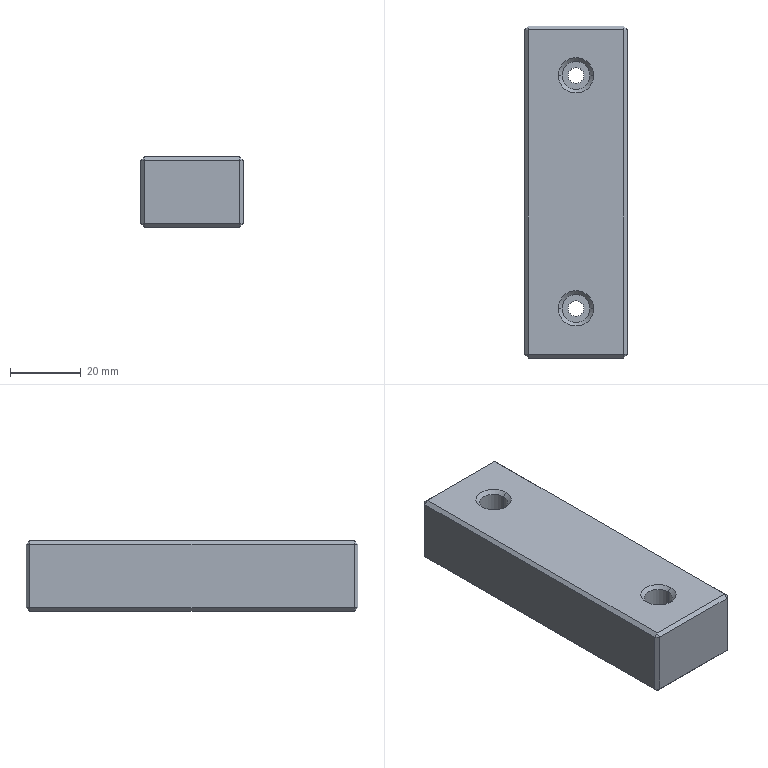Component | SolidWorks | CutterNylonPad-1 | 1 solid | 44 faces | box 29 x 94 x 20 mm | volume 52529 mm3 | plane 28 | cone 8 | cylinder 8 | commonest cylinder face diameters 8 x4 4.5 x4 | material 1060 Alloy
build123d program:
from build123d import *

# Parameters (mm, degrees)
SKETCH1_W                                          = 94
SKETCH1_H                                          = 20
BOSS_EXTRUDE1_DEPTH                                = 14.5
HOLE_SIZE_ACCORDING_TO_TYPE_OF_HEXAGON_D           = 4.5
HOLE_SIZE_ACCORDING_TO_TYPE_OF_HEXAGON_CBORE_D     = 8
HOLE_SIZE_ACCORDING_TO_TYPE_OF_HEXAGON_CBORE_DEPTH = 15
CHAMFER1_SIZE                                      = 1


with BuildPart() as part:
    # Sketch1 → Boss-Extrude1 (new, symmetric)
    with BuildSketch(Plane.XY):
        with Locations((0, -10)):
            Rectangle(SKETCH1_W, SKETCH1_H)
    extrude(amount=BOSS_EXTRUDE1_DEPTH, both=True)

    # Hole Size_ according to_Type of Hexagon (through all)
    with Locations(Plane(origin=(0, 0, 0), x_dir=(1, 0, 0), z_dir=(0, 1, 0))):
        with Locations((-33, 0), (33, 0)):
            CounterBoreHole(HOLE_SIZE_ACCORDING_TO_TYPE_OF_HEXAGON_D / 2, HOLE_SIZE_ACCORDING_TO_TYPE_OF_HEXAGON_CBORE_D / 2, HOLE_SIZE_ACCORDING_TO_TYPE_OF_HEXAGON_CBORE_DEPTH)

    # Chamfer1
    chamfer1_edges = [part.edges().sort_by_distance(p)[0] for p in [
        (47, -10, 14.5),
        (0, 0, 14.5),
        (29, 0, 0),
        (35.25, -20, 0),
        (-37, 0, 0),
        (-30.75, -20, 0),
        (-47, -10, 14.5),
        (0, 0, -14.5),
        (47, -10, -14.5),
        (0, -20, -14.5),
        (-47, -10, -14.5),
        (0, -20, 14.5),
        (-47, 0, 0),
        (47, 0, 0),
        (47, -20, 0),
        (-47, -20, 0),
    ]]
    chamfer(chamfer1_edges, length=CHAMFER1_SIZE)


solid = part.part

# Placed as in the assembly
solid = solid.moved(Location((-194.766, 347.264, -17), (90, -90, 0)))
STEP:
#1=COLOUR_RGB('',0.7922,0.8196,0.9333);
#2=FILL_AREA_STYLE_COLOUR('',#1);
#3=FILL_AREA_STYLE('',(#2));
#4=SURFACE_STYLE_FILL_AREA(#3);
#5=SURFACE_SIDE_STYLE('',(#4));
#6=SURFACE_STYLE_USAGE(.BOTH.,#5);
#7=PRESENTATION_STYLE_ASSIGNMENT((#6));
#8=CARTESIAN_POINT('',(-7.825,12.373,-0.7087));
#9=VERTEX_POINT('',#8);
#10=CARTESIAN_POINT('',(-7.51,12.373,-0.7087));
#11=VERTEX_POINT('',#10);
#12=CARTESIAN_POINT('',(-7.668,12.373,-0.7087));
#13=DIRECTION('',(-0.,-0.,1.));
#14=DIRECTION('',(-1.,0.,0.));
#15=AXIS2_PLACEMENT_3D('',#12,#13,#14);
#16=CIRCLE('',#15,0.1575);
#17=EDGE_CURVE('',#9,#11,#16,.T.);
#18=ORIENTED_EDGE('',*,*,#17,.F.);
#19=CARTESIAN_POINT('',(-7.865,12.373,-0.6693));
#20=VERTEX_POINT('',#19);
#21=CARTESIAN_POINT('',(-7.825,12.373,-0.7087));
#22=DIRECTION('',(-0.7071,0.,0.7071));
#23=VECTOR('',#22,39.37);
#24=LINE('',#21,#23);
#25=EDGE_CURVE('',#9,#20,#24,.T.);
#26=ORIENTED_EDGE('',*,*,#25,.T.);
#27=CARTESIAN_POINT('',(-7.471,12.373,-0.6693));
#28=VERTEX_POINT('',#27);
#29=CARTESIAN_POINT('',(-7.668,12.373,-0.6693));
#30=DIRECTION('',(0.,0.,-1.));
#31=DIRECTION('',(-1.,0.,0.));
#32=AXIS2_PLACEMENT_3D('',#29,#30,#31);
#33=CIRCLE('',#32,0.1969);
#34=EDGE_CURVE('',#28,#20,#33,.T.);
#35=ORIENTED_EDGE('',*,*,#34,.F.);
#36=CARTESIAN_POINT('',(-7.51,12.373,-0.7087));
#37=DIRECTION('',(0.7071,-0.,0.7071));
#38=VECTOR('',#37,39.37);
#39=LINE('',#36,#38);
#40=EDGE_CURVE('',#11,#28,#39,.T.);
#41=ORIENTED_EDGE('',*,*,#40,.F.);
#42=EDGE_LOOP('',(#18,#26,#35,#41));
#43=FACE_OUTER_BOUND('',#42,.T.);
#44=CARTESIAN_POINT('',(-7.668,12.373,-0.7087));
#45=DIRECTION('',(-0.,-0.,1.));
#46=DIRECTION('',(1.,0.,0.));
#47=AXIS2_PLACEMENT_3D('',#44,#45,#46);
#48=CONICAL_SURFACE('',#47,0.1575,0.7854);
#49=ADVANCED_FACE('',(#43),#48,.F.);
#50=CARTESIAN_POINT('',(-7.825,14.971,-0.7087));
#51=VERTEX_POINT('',#50);
#52=CARTESIAN_POINT('',(-7.51,14.971,-0.7087));
#53=VERTEX_POINT('',#52);
#54=CARTESIAN_POINT('',(-7.668,14.971,-0.7087));
#55=DIRECTION('',(-0.,-0.,1.));
#56=DIRECTION('',(-1.,0.,0.));
#57=AXIS2_PLACEMENT_3D('',#54,#55,#56);
#58=CIRCLE('',#57,0.1575);
#59=EDGE_CURVE('',#51,#53,#58,.T.);
#60=ORIENTED_EDGE('',*,*,#59,.F.);
#61=CARTESIAN_POINT('',(-7.865,14.971,-0.6693));
#62=VERTEX_POINT('',#61);
#63=CARTESIAN_POINT('',(-7.825,14.971,-0.7087));
#64=DIRECTION('',(-0.7071,0.,0.7071));
#65=VECTOR('',#64,39.37);
#66=LINE('',#63,#65);
#67=EDGE_CURVE('',#51,#62,#66,.T.);
#68=ORIENTED_EDGE('',*,*,#67,.T.);
#69=CARTESIAN_POINT('',(-7.471,14.971,-0.6693));
#70=VERTEX_POINT('',#69);
#71=CARTESIAN_POINT('',(-7.668,14.971,-0.6693));
#72=DIRECTION('',(0.,0.,-1.));
#73=DIRECTION('',(-1.,0.,0.));
#74=AXIS2_PLACEMENT_3D('',#71,#72,#73);
#75=CIRCLE('',#74,0.1969);
#76=EDGE_CURVE('',#70,#62,#75,.T.);
#77=ORIENTED_EDGE('',*,*,#76,.F.);
#78=CARTESIAN_POINT('',(-7.51,14.971,-0.7087));
#79=DIRECTION('',(0.7071,-0.,0.7071));
#80=VECTOR('',#79,39.37);
#81=LINE('',#78,#80);
#82=EDGE_CURVE('',#53,#70,#81,.T.);
#83=ORIENTED_EDGE('',*,*,#82,.F.);
#84=EDGE_LOOP('',(#60,#68,#77,#83));
#85=FACE_OUTER_BOUND('',#84,.T.);
#86=CARTESIAN_POINT('',(-7.668,14.971,-0.7087));
#87=DIRECTION('',(-0.,-0.,1.));
#88=DIRECTION('',(1.,0.,0.));
#89=AXIS2_PLACEMENT_3D('',#86,#87,#88);
#90=CONICAL_SURFACE('',#89,0.1575,0.7854);
#91=ADVANCED_FACE('',(#85),#90,.F.);
#92=CARTESIAN_POINT('',(-7.579,12.373,-1.417));
#93=VERTEX_POINT('',#92);
#94=CARTESIAN_POINT('',(-7.757,12.373,-1.417));
#95=VERTEX_POINT('',#94);
#96=CARTESIAN_POINT('',(-7.668,12.373,-1.417));
#97=DIRECTION('',(0.,0.,-1.));
#98=DIRECTION('',(1.,0.,0.));
#99=AXIS2_PLACEMENT_3D('',#96,#97,#98);
#100=CIRCLE('',#99,0.08858);
#101=EDGE_CURVE('',#93,#95,#100,.T.);
#102=ORIENTED_EDGE('',*,*,#101,.F.);
#103=CARTESIAN_POINT('',(-7.54,12.373,-1.457));
#104=VERTEX_POINT('',#103);
#105=CARTESIAN_POINT('',(-7.54,12.373,-1.457));
#106=DIRECTION('',(0.7071,0.,-0.7071));
#107=VECTOR('',#106,39.37);
#108=LINE('',#105,#107);
#109=EDGE_CURVE('',#93,#104,#108,.T.);
#110=ORIENTED_EDGE('',*,*,#109,.T.);
#111=CARTESIAN_POINT('',(-7.796,12.373,-1.457));
#112=VERTEX_POINT('',#111);
#113=CARTESIAN_POINT('',(-7.668,12.373,-1.457));
#114=DIRECTION('',(-0.,-0.,1.));
#115=DIRECTION('',(1.,0.,0.));
#116=AXIS2_PLACEMENT_3D('',#113,#114,#115);
#117=CIRCLE('',#116,0.128);
#118=EDGE_CURVE('',#112,#104,#117,.T.);
#119=ORIENTED_EDGE('',*,*,#118,.F.);
#120=CARTESIAN_POINT('',(-7.796,12.373,-1.457));
#121=DIRECTION('',(-0.7071,0.,-0.7071));
#122=VECTOR('',#121,39.37);
#123=LINE('',#120,#122);
#124=EDGE_CURVE('',#95,#112,#123,.T.);
#125=ORIENTED_EDGE('',*,*,#124,.F.);
#126=EDGE_LOOP('',(#102,#110,#119,#125));
#127=FACE_OUTER_BOUND('',#126,.T.);
#128=CARTESIAN_POINT('',(-7.668,12.373,-1.457));
#129=DIRECTION('',(0.,0.,-1.));
#130=DIRECTION('',(-1.,0.,0.));
#131=AXIS2_PLACEMENT_3D('',#128,#129,#130);
#132=CONICAL_SURFACE('',#131,0.128,0.7854);
#133=ADVANCED_FACE('',(#127),#132,.F.);
#134=CARTESIAN_POINT('',(-7.579,14.971,-1.417));
#135=VERTEX_POINT('',#134);
#136=CARTESIAN_POINT('',(-7.757,14.971,-1.417));
#137=VERTEX_POINT('',#136);
#138=CARTESIAN_POINT('',(-7.668,14.971,-1.417));
#139=DIRECTION('',(0.,0.,-1.));
#140=DIRECTION('',(1.,0.,0.));
#141=AXIS2_PLACEMENT_3D('',#138,#139,#140);
#142=CIRCLE('',#141,0.08858);
#143=EDGE_CURVE('',#135,#137,#142,.T.);
#144=ORIENTED_EDGE('',*,*,#143,.F.);
#145=CARTESIAN_POINT('',(-7.54,14.971,-1.457));
#146=VERTEX_POINT('',#145);
#147=CARTESIAN_POINT('',(-7.54,14.971,-1.457));
#148=DIRECTION('',(0.7071,0.,-0.7071));
#149=VECTOR('',#148,39.37);
#150=LINE('',#147,#149);
#151=EDGE_CURVE('',#135,#146,#150,.T.);
#152=ORIENTED_EDGE('',*,*,#151,.T.);
#153=CARTESIAN_POINT('',(-7.796,14.971,-1.457));
#154=VERTEX_POINT('',#153);
#155=CARTESIAN_POINT('',(-7.668,14.971,-1.457));
#156=DIRECTION('',(-0.,-0.,1.));
#157=DIRECTION('',(1.,0.,0.));
#158=AXIS2_PLACEMENT_3D('',#155,#156,#157);
#159=CIRCLE('',#158,0.128);
#160=EDGE_CURVE('',#154,#146,#159,.T.);
#161=ORIENTED_EDGE('',*,*,#160,.F.);
#162=CARTESIAN_POINT('',(-7.796,14.971,-1.457));
#163=DIRECTION('',(-0.7071,0.,-0.7071));
#164=VECTOR('',#163,39.37);
#165=LINE('',#162,#164);
#166=EDGE_CURVE('',#137,#154,#165,.T.);
#167=ORIENTED_EDGE('',*,*,#166,.F.);
#168=EDGE_LOOP('',(#144,#152,#161,#167));
#169=FACE_OUTER_BOUND('',#168,.T.);
#170=CARTESIAN_POINT('',(-7.668,14.971,-1.457));
#171=DIRECTION('',(0.,0.,-1.));
#172=DIRECTION('',(-1.,0.,0.));
#173=AXIS2_PLACEMENT_3D('',#170,#171,#172);
#174=CONICAL_SURFACE('',#173,0.128,0.7854);
#175=ADVANCED_FACE('',(#169),#174,.F.);
#176=CARTESIAN_POINT('',(-7.825,12.373,-1.26));
#177=VERTEX_POINT('',#176);
#178=CARTESIAN_POINT('',(-7.51,12.373,-1.26));
#179=VERTEX_POINT('',#178);
#180=CARTESIAN_POINT('',(-7.668,12.373,-1.26));
#181=DIRECTION('',(-0.,-0.,1.));
#182=DIRECTION('',(1.,0.,0.));
#183=AXIS2_PLACEMENT_3D('',#180,#181,#182);
#184=CIRCLE('',#183,0.1575);
#185=EDGE_CURVE('',#177,#179,#184,.T.);
#186=ORIENTED_EDGE('',*,*,#185,.F.);
#187=CARTESIAN_POINT('',(-7.825,12.373,-0.6693));
#188=DIRECTION('',(-0.,-0.,1.));
#189=VECTOR('',#188,39.37);
#190=LINE('',#187,#189);
#191=EDGE_CURVE('',#177,#9,#190,.T.);
#192=ORIENTED_EDGE('',*,*,#191,.T.);
#193=ORIENTED_EDGE('',*,*,#17,.T.);
#194=CARTESIAN_POINT('',(-7.51,12.373,-0.6693));
#195=DIRECTION('',(-0.,-0.,1.));
#196=VECTOR('',#195,39.37);
#197=LINE('',#194,#196);
#198=EDGE_CURVE('',#179,#11,#197,.T.);
#199=ORIENTED_EDGE('',*,*,#198,.F.);
#200=EDGE_LOOP('',(#186,#192,#193,#199));
#201=FACE_OUTER_BOUND('',#200,.T.);
#202=CARTESIAN_POINT('',(-7.668,12.373,-0.6693));
#203=DIRECTION('',(-0.,-0.,1.));
#204=DIRECTION('',(1.,0.,0.));
#205=AXIS2_PLACEMENT_3D('',#202,#203,#204);
#206=CYLINDRICAL_SURFACE('',#205,0.1575);
#207=ADVANCED_FACE('',(#201),#206,.F.);
#208=ORIENTED_EDGE('',*,*,#101,.T.);
#209=CARTESIAN_POINT('',(-7.757,12.373,-1.26));
#210=VERTEX_POINT('',#209);
#211=CARTESIAN_POINT('',(-7.757,12.373,-0.6693));
#212=DIRECTION('',(-0.,-0.,1.));
#213=VECTOR('',#212,39.37);
#214=LINE('',#211,#213);
#215=EDGE_CURVE('',#95,#210,#214,.T.);
#216=ORIENTED_EDGE('',*,*,#215,.T.);
#217=CARTESIAN_POINT('',(-7.579,12.373,-1.26));
#218=VERTEX_POINT('',#217);
#219=CARTESIAN_POINT('',(-7.668,12.373,-1.26));
#220=DIRECTION('',(-0.,-0.,1.));
#221=DIRECTION('',(1.,0.,0.));
#222=AXIS2_PLACEMENT_3D('',#219,#220,#221);
#223=CIRCLE('',#222,0.08858);
#224=EDGE_CURVE('',#210,#218,#223,.T.);
#225=ORIENTED_EDGE('',*,*,#224,.T.);
#226=CARTESIAN_POINT('',(-7.579,12.373,-0.6693));
#227=DIRECTION('',(-0.,-0.,1.));
#228=VECTOR('',#227,39.37);
#229=LINE('',#226,#228);
#230=EDGE_CURVE('',#93,#218,#229,.T.);
#231=ORIENTED_EDGE('',*,*,#230,.F.);
#232=EDGE_LOOP('',(#208,#216,#225,#231));
#233=FACE_OUTER_BOUND('',#232,.T.);
#234=CARTESIAN_POINT('',(-7.668,12.373,-0.6693));
#235=DIRECTION('',(-0.,-0.,1.));
#236=DIRECTION('',(1.,0.,0.));
#237=AXIS2_PLACEMENT_3D('',#234,#235,#236);
#238=CYLINDRICAL_SURFACE('',#237,0.08858);
#239=ADVANCED_FACE('',(#233),#238,.F.);
#240=CARTESIAN_POINT('',(-7.825,14.971,-1.26));
#241=VERTEX_POINT('',#240);
#242=CARTESIAN_POINT('',(-7.51,14.971,-1.26));
#243=VERTEX_POINT('',#242);
#244=CARTESIAN_POINT('',(-7.668,14.971,-1.26));
#245=DIRECTION('',(-0.,-0.,1.));
#246=DIRECTION('',(1.,0.,0.));
#247=AXIS2_PLACEMENT_3D('',#244,#245,#246);
#248=CIRCLE('',#247,0.1575);
#249=EDGE_CURVE('',#241,#243,#248,.T.);
#250=ORIENTED_EDGE('',*,*,#249,.F.);
#251=CARTESIAN_POINT('',(-7.825,14.971,-0.6693));
#252=DIRECTION('',(-0.,-0.,1.));
#253=VECTOR('',#252,39.37);
#254=LINE('',#251,#253);
#255=EDGE_CURVE('',#241,#51,#254,.T.);
#256=ORIENTED_EDGE('',*,*,#255,.T.);
#257=ORIENTED_EDGE('',*,*,#59,.T.);
#258=CARTESIAN_POINT('',(-7.51,14.971,-0.6693));
#259=DIRECTION('',(-0.,-0.,1.));
#260=VECTOR('',#259,39.37);
#261=LINE('',#258,#260);
#262=EDGE_CURVE('',#243,#53,#261,.T.);
#263=ORIENTED_EDGE('',*,*,#262,.F.);
#264=EDGE_LOOP('',(#250,#256,#257,#263));
#265=FACE_OUTER_BOUND('',#264,.T.);
#266=CARTESIAN_POINT('',(-7.668,14.971,-0.6693));
#267=DIRECTION('',(-0.,-0.,1.));
#268=DIRECTION('',(1.,0.,0.));
#269=AXIS2_PLACEMENT_3D('',#266,#267,#268);
#270=CYLINDRICAL_SURFACE('',#269,0.1575);
#271=ADVANCED_FACE('',(#265),#270,.F.);
#272=ORIENTED_EDGE('',*,*,#143,.T.);
#273=CARTESIAN_POINT('',(-7.757,14.971,-1.26));
#274=VERTEX_POINT('',#273);
#275=CARTESIAN_POINT('',(-7.757,14.971,-0.6693));
#276=DIRECTION('',(-0.,-0.,1.));
#277=VECTOR('',#276,39.37);
#278=LINE('',#275,#277);
#279=EDGE_CURVE('',#137,#274,#278,.T.);
#280=ORIENTED_EDGE('',*,*,#279,.T.);
#281=CARTESIAN_POINT('',(-7.579,14.971,-1.26));
#282=VERTEX_POINT('',#281);
#283=CARTESIAN_POINT('',(-7.668,14.971,-1.26));
#284=DIRECTION('',(-0.,-0.,1.));
#285=DIRECTION('',(1.,0.,0.));
#286=AXIS2_PLACEMENT_3D('',#283,#284,#285);
#287=CIRCLE('',#286,0.08858);
#288=EDGE_CURVE('',#274,#282,#287,.T.);
#289=ORIENTED_EDGE('',*,*,#288,.T.);
#290=CARTESIAN_POINT('',(-7.579,14.971,-0.6693));
#291=DIRECTION('',(-0.,-0.,1.));
#292=VECTOR('',#291,39.37);
#293=LINE('',#290,#292);
#294=EDGE_CURVE('',#135,#282,#293,.T.);
#295=ORIENTED_EDGE('',*,*,#294,.F.);
#296=EDGE_LOOP('',(#272,#280,#289,#295));
#297=FACE_OUTER_BOUND('',#296,.T.);
#298=CARTESIAN_POINT('',(-7.668,14.971,-0.6693));
#299=DIRECTION('',(-0.,-0.,1.));
#300=DIRECTION('',(1.,0.,0.));
#301=AXIS2_PLACEMENT_3D('',#298,#299,#300);
#302=CYLINDRICAL_SURFACE('',#301,0.08858);
#303=ADVANCED_FACE('',(#297),#302,.F.);
#304=CARTESIAN_POINT('',(-8.199,11.821,-0.7087));
#305=VERTEX_POINT('',#304);
#306=CARTESIAN_POINT('',(-8.199,11.821,-1.417));
#307=VERTEX_POINT('',#306);
#308=CARTESIAN_POINT('',(-8.199,11.821,-0.6693));
#309=DIRECTION('',(0.,0.,-1.));
#310=VECTOR('',#309,39.37);
#311=LINE('',#308,#310);
#312=EDGE_CURVE('',#305,#307,#311,.T.);
#313=ORIENTED_EDGE('',*,*,#312,.T.);
#314=CARTESIAN_POINT('',(-7.136,11.821,-1.417));
#315=VERTEX_POINT('',#314);
#316=CARTESIAN_POINT('',(-7.097,11.821,-1.417));
#317=DIRECTION('',(1.,0.,0.));
#318=VECTOR('',#317,39.37);
#319=LINE('',#316,#318);
#320=EDGE_CURVE('',#307,#315,#319,.T.);
#321=ORIENTED_EDGE('',*,*,#320,.T.);
#322=CARTESIAN_POINT('',(-7.136,11.821,-0.7087));
#323=VERTEX_POINT('',#322);
#324=CARTESIAN_POINT('',(-7.136,11.821,-0.6693));
#325=DIRECTION('',(-0.,-0.,1.));
#326=VECTOR('',#325,39.37);
#327=LINE('',#324,#326);
#328=EDGE_CURVE('',#315,#323,#327,.T.);
#329=ORIENTED_EDGE('',*,*,#328,.T.);
#330=CARTESIAN_POINT('',(-7.097,11.821,-0.7087));
#331=DIRECTION('',(-1.,-0.,-0.));
#332=VECTOR('',#331,39.37);
#333=LINE('',#330,#332);
#334=EDGE_CURVE('',#323,#305,#333,.T.);
#335=ORIENTED_EDGE('',*,*,#334,.T.);
#336=EDGE_LOOP('',(#313,#321,#329,#335));
#337=FACE_OUTER_BOUND('',#336,.T.);
#338=CARTESIAN_POINT('',(-7.097,11.821,-0.6693));
#339=DIRECTION('',(-0.,1.,0.));
#340=DIRECTION('',(-1.,-0.,-0.));
#341=AXIS2_PLACEMENT_3D('',#338,#339,#340);
#342=PLANE('',#341);
#343=ADVANCED_FACE('',(#337),#342,.F.);
#344=ORIENTED_EDGE('',*,*,#160,.T.);
#345=CARTESIAN_POINT('',(-7.668,14.971,-1.457));
#346=DIRECTION('',(-0.,-0.,1.));
#347=DIRECTION('',(1.,0.,0.));
#348=AXIS2_PLACEMENT_3D('',#345,#346,#347);
#349=CIRCLE('',#348,0.128);
#350=EDGE_CURVE('',#146,#154,#349,.T.);
#351=ORIENTED_EDGE('',*,*,#350,.T.);
#352=EDGE_LOOP('',(#344,#351));
#353=FACE_BOUND('',#352,.T.);
#354=ORIENTED_EDGE('',*,*,#118,.T.);
#355=CARTESIAN_POINT('',(-7.668,12.373,-1.457));
#356=DIRECTION('',(-0.,-0.,1.));
#357=DIRECTION('',(1.,0.,0.));
#358=AXIS2_PLACEMENT_3D('',#355,#356,#357);
#359=CIRCLE('',#358,0.128);
#360=EDGE_CURVE('',#104,#112,#359,.T.);
#361=ORIENTED_EDGE('',*,*,#360,.T.);
#362=EDGE_LOOP('',(#354,#361));
#363=FACE_BOUND('',#362,.T.);
#364=CARTESIAN_POINT('',(-7.136,15.483,-1.457));
#365=VERTEX_POINT('',#364);
#366=CARTESIAN_POINT('',(-7.136,11.861,-1.457));
#367=VERTEX_POINT('',#366);
#368=CARTESIAN_POINT('',(-7.136,11.821,-1.457));
#369=DIRECTION('',(0.,-1.,-0.));
#370=VECTOR('',#369,39.37);
#371=LINE('',#368,#370);
#372=EDGE_CURVE('',#365,#367,#371,.T.);
#373=ORIENTED_EDGE('',*,*,#372,.T.);
#374=CARTESIAN_POINT('',(-8.199,11.861,-1.457));
#375=VERTEX_POINT('',#374);
#376=CARTESIAN_POINT('',(-7.097,11.861,-1.457));
#377=DIRECTION('',(-1.,-0.,-0.));
#378=VECTOR('',#377,39.37);
#379=LINE('',#376,#378);
#380=EDGE_CURVE('',#367,#375,#379,.T.);
#381=ORIENTED_EDGE('',*,*,#380,.T.);
#382=CARTESIAN_POINT('',(-8.199,15.483,-1.457));
#383=VERTEX_POINT('',#382);
#384=CARTESIAN_POINT('',(-8.199,11.821,-1.457));
#385=DIRECTION('',(-0.,1.,0.));
#386=VECTOR('',#385,39.37);
#387=LINE('',#384,#386);
#388=EDGE_CURVE('',#375,#383,#387,.T.);
#389=ORIENTED_EDGE('',*,*,#388,.T.);
#390=CARTESIAN_POINT('',(-7.097,15.483,-1.457));
#391=DIRECTION('',(1.,0.,0.));
#392=VECTOR('',#391,39.37);
#393=LINE('',#390,#392);
#394=EDGE_CURVE('',#383,#365,#393,.T.);
#395=ORIENTED_EDGE('',*,*,#394,.T.);
#396=EDGE_LOOP('',(#373,#381,#389,#395));
#397=FACE_OUTER_BOUND('',#396,.T.);
#398=CARTESIAN_POINT('',(-7.097,11.821,-1.457));
#399=DIRECTION('',(-0.,-0.,1.));
#400=DIRECTION('',(1.,0.,0.));
#401=AXIS2_PLACEMENT_3D('',#398,#399,#400);
#402=PLANE('',#401);
#403=ADVANCED_FACE('',(#353,#363,#397),#402,.F.);
#404=CARTESIAN_POINT('',(-7.136,15.522,-0.7087));
#405=VERTEX_POINT('',#404);
#406=CARTESIAN_POINT('',(-7.136,15.522,-1.417));
#407=VERTEX_POINT('',#406);
#408=CARTESIAN_POINT('',(-7.136,15.522,-1.457));
#409=DIRECTION('',(0.,0.,-1.));
#410=VECTOR('',#409,39.37);
#411=LINE('',#408,#410);
#412=EDGE_CURVE('',#405,#407,#411,.T.);
#413=ORIENTED_EDGE('',*,*,#412,.T.);
#414=CARTESIAN_POINT('',(-8.199,15.522,-1.417));
#415=VERTEX_POINT('',#414);
#416=CARTESIAN_POINT('',(-7.097,15.522,-1.417));
#417=DIRECTION('',(-1.,-0.,-0.));
#418=VECTOR('',#417,39.37);
#419=LINE('',#416,#418);
#420=EDGE_CURVE('',#407,#415,#419,.T.);
#421=ORIENTED_EDGE('',*,*,#420,.T.);
#422=CARTESIAN_POINT('',(-8.199,15.522,-0.7087));
#423=VERTEX_POINT('',#422);
#424=CARTESIAN_POINT('',(-8.199,15.522,-0.6693));
#425=DIRECTION('',(-0.,-0.,1.));
#426=VECTOR('',#425,39.37);
#427=LINE('',#424,#426);
#428=EDGE_CURVE('',#415,#423,#427,.T.);
#429=ORIENTED_EDGE('',*,*,#428,.T.);
#430=CARTESIAN_POINT('',(-7.097,15.522,-0.7087));
#431=DIRECTION('',(1.,0.,0.));
#432=VECTOR('',#431,39.37);
#433=LINE('',#430,#432);
#434=EDGE_CURVE('',#423,#405,#433,.T.);
#435=ORIENTED_EDGE('',*,*,#434,.T.);
#436=EDGE_LOOP('',(#413,#421,#429,#435));
#437=FACE_OUTER_BOUND('',#436,.T.);
#438=CARTESIAN_POINT('',(-7.097,15.522,-0.6693));
#439=DIRECTION('',(0.,-1.,-0.));
#440=DIRECTION('',(1.,0.,0.));
#441=AXIS2_PLACEMENT_3D('',#438,#439,#440);
#442=PLANE('',#441);
#443=ADVANCED_FACE('',(#437),#442,.F.);
#444=CARTESIAN_POINT('',(-7.136,11.861,-0.6693));
#445=VERTEX_POINT('',#444);
#446=CARTESIAN_POINT('',(-7.136,15.483,-0.6693));
#447=VERTEX_POINT('',#446);
#448=CARTESIAN_POINT('',(-7.136,15.522,-0.6693));
#449=DIRECTION('',(-0.,1.,0.));
#450=VECTOR('',#449,39.37);
#451=LINE('',#448,#450);
#452=EDGE_CURVE('',#445,#447,#451,.T.);
#453=ORIENTED_EDGE('',*,*,#452,.T.);
#454=CARTESIAN_POINT('',(-8.199,15.483,-0.6693));
#455=VERTEX_POINT('',#454);
#456=CARTESIAN_POINT('',(-7.097,15.483,-0.6693));
#457=DIRECTION('',(-1.,-0.,-0.));
#458=VECTOR('',#457,39.37);
#459=LINE('',#456,#458);
#460=EDGE_CURVE('',#447,#455,#459,.T.);
#461=ORIENTED_EDGE('',*,*,#460,.T.);
#462=CARTESIAN_POINT('',(-8.199,11.861,-0.6693));
#463=VERTEX_POINT('',#462);
#464=CARTESIAN_POINT('',(-8.199,11.821,-0.6693));
#465=DIRECTION('',(0.,-1.,-0.));
#466=VECTOR('',#465,39.37);
#467=LINE('',#464,#466);
#468=EDGE_CURVE('',#455,#463,#467,.T.);
#469=ORIENTED_EDGE('',*,*,#468,.T.);
#470=CARTESIAN_POINT('',(-7.097,11.861,-0.6693));
#471=DIRECTION('',(1.,0.,0.));
#472=VECTOR('',#471,39.37);
#473=LINE('',#470,#472);
#474=EDGE_CURVE('',#463,#445,#473,.T.);
#475=ORIENTED_EDGE('',*,*,#474,.T.);
#476=EDGE_LOOP('',(#453,#461,#469,#475));
#477=FACE_OUTER_BOUND('',#476,.T.);
#478=ORIENTED_EDGE('',*,*,#76,.T.);
#479=CARTESIAN_POINT('',(-7.668,14.971,-0.6693));
#480=DIRECTION('',(0.,0.,-1.));
#481=DIRECTION('',(-1.,0.,0.));
#482=AXIS2_PLACEMENT_3D('',#479,#480,#481);
#483=CIRCLE('',#482,0.1969);
#484=EDGE_CURVE('',#62,#70,#483,.T.);
#485=ORIENTED_EDGE('',*,*,#484,.T.);
#486=EDGE_LOOP('',(#478,#485));
#487=FACE_BOUND('',#486,.T.);
#488=ORIENTED_EDGE('',*,*,#34,.T.);
#489=CARTESIAN_POINT('',(-7.668,12.373,-0.6693));
#490=DIRECTION('',(0.,0.,-1.));
#491=DIRECTION('',(-1.,0.,0.));
#492=AXIS2_PLACEMENT_3D('',#489,#490,#491);
#493=CIRCLE('',#492,0.1969);
#494=EDGE_CURVE('',#20,#28,#493,.T.);
#495=ORIENTED_EDGE('',*,*,#494,.T.);
#496=EDGE_LOOP('',(#488,#495));
#497=FACE_BOUND('',#496,.T.);
#498=CARTESIAN_POINT('',(-7.097,11.821,-0.6693));
#499=DIRECTION('',(0.,0.,-1.));
#500=DIRECTION('',(-1.,-0.,-0.));
#501=AXIS2_PLACEMENT_3D('',#498,#499,#500);
#502=PLANE('',#501);
#503=ADVANCED_FACE('',(#477,#487,#497),#502,.F.);
#504=CARTESIAN_POINT('',(-7.097,15.483,-0.7087));
#505=VERTEX_POINT('',#504);
#506=CARTESIAN_POINT('',(-7.097,11.861,-0.7087));
#507=VERTEX_POINT('',#506);
#508=CARTESIAN_POINT('',(-7.097,11.821,-0.7087));
#509=DIRECTION('',(0.,-1.,-0.));
#510=VECTOR('',#509,39.37);
#511=LINE('',#508,#510);
#512=EDGE_CURVE('',#505,#507,#511,.T.);
#513=ORIENTED_EDGE('',*,*,#512,.T.);
#514=CARTESIAN_POINT('',(-7.097,11.861,-1.417));
#515=VERTEX_POINT('',#514);
#516=CARTESIAN_POINT('',(-7.097,11.861,-1.457));
#517=DIRECTION('',(0.,0.,-1.));
#518=VECTOR('',#517,39.37);
#519=LINE('',#516,#518);
#520=EDGE_CURVE('',#507,#515,#519,.T.);
#521=ORIENTED_EDGE('',*,*,#520,.T.);
#522=CARTESIAN_POINT('',(-7.097,15.483,-1.417));
#523=VERTEX_POINT('',#522);
#524=CARTESIAN_POINT('',(-7.097,15.522,-1.417));
#525=DIRECTION('',(-0.,1.,0.));
#526=VECTOR('',#525,39.37);
#527=LINE('',#524,#526);
#528=EDGE_CURVE('',#515,#523,#527,.T.);
#529=ORIENTED_EDGE('',*,*,#528,.T.);
#530=CARTESIAN_POINT('',(-7.097,15.483,-0.6693));
#531=DIRECTION('',(-0.,-0.,1.));
#532=VECTOR('',#531,39.37);
#533=LINE('',#530,#532);
#534=EDGE_CURVE('',#523,#505,#533,.T.);
#535=ORIENTED_EDGE('',*,*,#534,.T.);
#536=EDGE_LOOP('',(#513,#521,#529,#535));
#537=FACE_OUTER_BOUND('',#536,.T.);
#538=CARTESIAN_POINT('',(-7.097,13.672,-0.6693));
#539=DIRECTION('',(1.,0.,0.));
#540=DIRECTION('',(-0.,1.,0.));
#541=AXIS2_PLACEMENT_3D('',#538,#539,#540);
#542=PLANE('',#541);
#543=ADVANCED_FACE('',(#537),#542,.T.);
#544=CARTESIAN_POINT('',(-8.239,15.483,-1.417));
#545=VERTEX_POINT('',#544);
#546=CARTESIAN_POINT('',(-8.239,11.861,-1.417));
#547=VERTEX_POINT('',#546);
#548=CARTESIAN_POINT('',(-8.239,13.672,-1.417));
#549=DIRECTION('',(0.,-1.,-0.));
#550=VECTOR('',#549,39.37);
#551=LINE('',#548,#550);
#552=EDGE_CURVE('',#545,#547,#551,.T.);
#553=ORIENTED_EDGE('',*,*,#552,.T.);
#554=CARTESIAN_POINT('',(-8.239,11.861,-0.7087));
#555=VERTEX_POINT('',#554);
#556=CARTESIAN_POINT('',(-8.239,11.861,-0.6693));
#557=DIRECTION('',(-0.,-0.,1.));
#558=VECTOR('',#557,39.37);
#559=LINE('',#556,#558);
#560=EDGE_CURVE('',#547,#555,#559,.T.);
#561=ORIENTED_EDGE('',*,*,#560,.T.);
#562=CARTESIAN_POINT('',(-8.239,15.483,-0.7087));
#563=VERTEX_POINT('',#562);
#564=CARTESIAN_POINT('',(-8.239,13.672,-0.7087));
#565=DIRECTION('',(-0.,1.,0.));
#566=VECTOR('',#565,39.37);
#567=LINE('',#564,#566);
#568=EDGE_CURVE('',#555,#563,#567,.T.);
#569=ORIENTED_EDGE('',*,*,#568,.T.);
#570=CARTESIAN_POINT('',(-8.239,15.483,-0.6693));
#571=DIRECTION('',(0.,0.,-1.));
#572=VECTOR('',#571,39.37);
#573=LINE('',#570,#572);
#574=EDGE_CURVE('',#563,#545,#573,.T.);
#575=ORIENTED_EDGE('',*,*,#574,.T.);
#576=EDGE_LOOP('',(#553,#561,#569,#575));
#577=FACE_OUTER_BOUND('',#576,.T.);
#578=CARTESIAN_POINT('',(-8.239,13.672,-0.6693));
#579=DIRECTION('',(1.,0.,0.));
#580=DIRECTION('',(-0.,1.,0.));
#581=AXIS2_PLACEMENT_3D('',#578,#579,#580);
#582=PLANE('',#581);
#583=ADVANCED_FACE('',(#577),#582,.F.);
#584=ORIENTED_EDGE('',*,*,#279,.F.);
#585=CARTESIAN_POINT('',(-7.668,14.971,-1.417));
#586=DIRECTION('',(0.,0.,-1.));
#587=DIRECTION('',(1.,0.,0.));
#588=AXIS2_PLACEMENT_3D('',#585,#586,#587);
#589=CIRCLE('',#588,0.08858);
#590=EDGE_CURVE('',#137,#135,#589,.T.);
#591=ORIENTED_EDGE('',*,*,#590,.T.);
#592=ORIENTED_EDGE('',*,*,#294,.T.);
#593=CARTESIAN_POINT('',(-7.668,14.971,-1.26));
#594=DIRECTION('',(-0.,-0.,1.));
#595=DIRECTION('',(1.,0.,0.));
#596=AXIS2_PLACEMENT_3D('',#593,#594,#595);
#597=CIRCLE('',#596,0.08858);
#598=EDGE_CURVE('',#282,#274,#597,.T.);
#599=ORIENTED_EDGE('',*,*,#598,.T.);
#600=EDGE_LOOP('',(#584,#591,#592,#599));
#601=FACE_OUTER_BOUND('',#600,.T.);
#602=CARTESIAN_POINT('',(-7.668,14.971,-0.6693));
#603=DIRECTION('',(-0.,-0.,1.));
#604=DIRECTION('',(1.,0.,0.));
#605=AXIS2_PLACEMENT_3D('',#602,#603,#604);
#606=CYLINDRICAL_SURFACE('',#605,0.08858);
#607=ADVANCED_FACE('',(#601),#606,.F.);
#608=ORIENTED_EDGE('',*,*,#598,.F.);
#609=ORIENTED_EDGE('',*,*,#288,.F.);
#610=EDGE_LOOP('',(#608,#609));
#611=FACE_BOUND('',#610,.T.);
#612=CARTESIAN_POINT('',(-7.668,14.971,-1.26));
#613=DIRECTION('',(-0.,-0.,1.));
#614=DIRECTION('',(1.,0.,0.));
#615=AXIS2_PLACEMENT_3D('',#612,#613,#614);
#616=CIRCLE('',#615,0.1575);
#617=EDGE_CURVE('',#243,#241,#616,.T.);
#618=ORIENTED_EDGE('',*,*,#617,.T.);
#619=ORIENTED_EDGE('',*,*,#249,.T.);
#620=EDGE_LOOP('',(#618,#619));
#621=FACE_OUTER_BOUND('',#620,.T.);
#622=CARTESIAN_POINT('',(-7.668,15.06,-1.26));
#623=DIRECTION('',(0.,0.,-1.));
#624=DIRECTION('',(-1.,-0.,-0.));
#625=AXIS2_PLACEMENT_3D('',#622,#623,#624);
#626=PLANE('',#625);
#627=ADVANCED_FACE('',(#611,#621),#626,.F.);
#628=ORIENTED_EDGE('',*,*,#255,.F.);
#629=ORIENTED_EDGE('',*,*,#617,.F.);
#630=ORIENTED_EDGE('',*,*,#262,.T.);
#631=CARTESIAN_POINT('',(-7.668,14.971,-0.7087));
#632=DIRECTION('',(-0.,-0.,1.));
#633=DIRECTION('',(-1.,0.,0.));
#634=AXIS2_PLACEMENT_3D('',#631,#632,#633);
#635=CIRCLE('',#634,0.1575);
#636=EDGE_CURVE('',#53,#51,#635,.T.);
#637=ORIENTED_EDGE('',*,*,#636,.T.);
#638=EDGE_LOOP('',(#628,#629,#630,#637));
#639=FACE_OUTER_BOUND('',#638,.T.);
#640=CARTESIAN_POINT('',(-7.668,14.971,-0.6693));
#641=DIRECTION('',(-0.,-0.,1.));
#642=DIRECTION('',(1.,0.,0.));
#643=AXIS2_PLACEMENT_3D('',#640,#641,#642);
#644=CYLINDRICAL_SURFACE('',#643,0.1575);
#645=ADVANCED_FACE('',(#639),#644,.F.);
#646=ORIENTED_EDGE('',*,*,#215,.F.);
#647=CARTESIAN_POINT('',(-7.668,12.373,-1.417));
#648=DIRECTION('',(0.,0.,-1.));
#649=DIRECTION('',(1.,0.,0.));
#650=AXIS2_PLACEMENT_3D('',#647,#648,#649);
#651=CIRCLE('',#650,0.08858);
#652=EDGE_CURVE('',#95,#93,#651,.T.);
#653=ORIENTED_EDGE('',*,*,#652,.T.);
#654=ORIENTED_EDGE('',*,*,#230,.T.);
#655=CARTESIAN_POINT('',(-7.668,12.373,-1.26));
#656=DIRECTION('',(-0.,-0.,1.));
#657=DIRECTION('',(1.,0.,0.));
#658=AXIS2_PLACEMENT_3D('',#655,#656,#657);
#659=CIRCLE('',#658,0.08858);
#660=EDGE_CURVE('',#218,#210,#659,.T.);
#661=ORIENTED_EDGE('',*,*,#660,.T.);
#662=EDGE_LOOP('',(#646,#653,#654,#661));
#663=FACE_OUTER_BOUND('',#662,.T.);
#664=CARTESIAN_POINT('',(-7.668,12.373,-0.6693));
#665=DIRECTION('',(-0.,-0.,1.));
#666=DIRECTION('',(1.,0.,0.));
#667=AXIS2_PLACEMENT_3D('',#664,#665,#666);
#668=CYLINDRICAL_SURFACE('',#667,0.08858);
#669=ADVANCED_FACE('',(#663),#668,.F.);
#670=ORIENTED_EDGE('',*,*,#660,.F.);
#671=ORIENTED_EDGE('',*,*,#224,.F.);
#672=EDGE_LOOP('',(#670,#671));
#673=FACE_BOUND('',#672,.T.);
#674=CARTESIAN_POINT('',(-7.668,12.373,-1.26));
#675=DIRECTION('',(-0.,-0.,1.));
#676=DIRECTION('',(1.,0.,0.));
#677=AXIS2_PLACEMENT_3D('',#674,#675,#676);
#678=CIRCLE('',#677,0.1575);
#679=EDGE_CURVE('',#179,#177,#678,.T.);
#680=ORIENTED_EDGE('',*,*,#679,.T.);
#681=ORIENTED_EDGE('',*,*,#185,.T.);
#682=EDGE_LOOP('',(#680,#681));
#683=FACE_OUTER_BOUND('',#682,.T.);
#684=CARTESIAN_POINT('',(-7.668,12.461,-1.26));
#685=DIRECTION('',(0.,0.,-1.));
#686=DIRECTION('',(-1.,-0.,-0.));
#687=AXIS2_PLACEMENT_3D('',#684,#685,#686);
#688=PLANE('',#687);
#689=ADVANCED_FACE('',(#673,#683),#688,.F.);
#690=ORIENTED_EDGE('',*,*,#191,.F.);
#691=ORIENTED_EDGE('',*,*,#679,.F.);
#692=ORIENTED_EDGE('',*,*,#198,.T.);
#693=CARTESIAN_POINT('',(-7.668,12.373,-0.7087));
#694=DIRECTION('',(-0.,-0.,1.));
#695=DIRECTION('',(-1.,0.,0.));
#696=AXIS2_PLACEMENT_3D('',#693,#694,#695);
#697=CIRCLE('',#696,0.1575);
#698=EDGE_CURVE('',#11,#9,#697,.T.);
#699=ORIENTED_EDGE('',*,*,#698,.T.);
#700=EDGE_LOOP('',(#690,#691,#692,#699));
#701=FACE_OUTER_BOUND('',#700,.T.);
#702=CARTESIAN_POINT('',(-7.668,12.373,-0.6693));
#703=DIRECTION('',(-0.,-0.,1.));
#704=DIRECTION('',(1.,0.,0.));
#705=AXIS2_PLACEMENT_3D('',#702,#703,#704);
#706=CYLINDRICAL_SURFACE('',#705,0.1575);
#707=ADVANCED_FACE('',(#701),#706,.F.);
#708=ORIENTED_EDGE('',*,*,#151,.F.);
#709=ORIENTED_EDGE('',*,*,#590,.F.);
#710=ORIENTED_EDGE('',*,*,#166,.T.);
#711=ORIENTED_EDGE('',*,*,#350,.F.);
#712=EDGE_LOOP('',(#708,#709,#710,#711));
#713=FACE_OUTER_BOUND('',#712,.T.);
#714=CARTESIAN_POINT('',(-7.668,14.971,-1.457));
#715=DIRECTION('',(0.,0.,-1.));
#716=DIRECTION('',(-1.,0.,0.));
#717=AXIS2_PLACEMENT_3D('',#714,#715,#716);
#718=CONICAL_SURFACE('',#717,0.128,0.7854);
#719=ADVANCED_FACE('',(#713),#718,.F.);
#720=ORIENTED_EDGE('',*,*,#109,.F.);
#721=ORIENTED_EDGE('',*,*,#652,.F.);
#722=ORIENTED_EDGE('',*,*,#124,.T.);
#723=ORIENTED_EDGE('',*,*,#360,.F.);
#724=EDGE_LOOP('',(#720,#721,#722,#723));
#725=FACE_OUTER_BOUND('',#724,.T.);
#726=CARTESIAN_POINT('',(-7.668,12.373,-1.457));
#727=DIRECTION('',(0.,0.,-1.));
#728=DIRECTION('',(-1.,0.,0.));
#729=AXIS2_PLACEMENT_3D('',#726,#727,#728);
#730=CONICAL_SURFACE('',#729,0.128,0.7854);
#731=ADVANCED_FACE('',(#725),#730,.F.);
#732=CARTESIAN_POINT('',(-8.199,15.522,-0.7087));
#733=DIRECTION('',(-0.7071,-0.7071,-0.));
#734=VECTOR('',#733,39.37);
#735=LINE('',#732,#734);
#736=EDGE_CURVE('',#423,#563,#735,.T.);
#737=ORIENTED_EDGE('',*,*,#736,.F.);
#738=ORIENTED_EDGE('',*,*,#428,.F.);
#739=CARTESIAN_POINT('',(-8.219,15.503,-1.417));
#740=DIRECTION('',(0.7071,0.7071,-0.));
#741=VECTOR('',#740,39.37);
#742=LINE('',#739,#741);
#743=EDGE_CURVE('',#545,#415,#742,.T.);
#744=ORIENTED_EDGE('',*,*,#743,.F.);
#745=ORIENTED_EDGE('',*,*,#574,.F.);
#746=EDGE_LOOP('',(#737,#738,#744,#745));
#747=FACE_OUTER_BOUND('',#746,.T.);
#748=CARTESIAN_POINT('',(-8.199,15.522,-0.6693));
#749=DIRECTION('',(0.7071,-0.7071,-0.));
#750=DIRECTION('',(-0.,-0.,1.));
#751=AXIS2_PLACEMENT_3D('',#748,#749,#750);
#752=PLANE('',#751);
#753=ADVANCED_FACE('',(#747),#752,.F.);
#754=CARTESIAN_POINT('',(-8.199,15.522,-0.7087));
#755=DIRECTION('',(-0.,-0.7071,0.7071));
#756=VECTOR('',#755,39.37);
#757=LINE('',#754,#756);
#758=EDGE_CURVE('',#423,#455,#757,.T.);
#759=ORIENTED_EDGE('',*,*,#758,.F.);
#760=ORIENTED_EDGE('',*,*,#736,.T.);
#761=CARTESIAN_POINT('',(-8.219,15.483,-0.689));
#762=DIRECTION('',(-0.7071,-0.,-0.7071));
#763=VECTOR('',#762,39.37);
#764=LINE('',#761,#763);
#765=EDGE_CURVE('',#455,#563,#764,.T.);
#766=ORIENTED_EDGE('',*,*,#765,.F.);
#767=EDGE_LOOP('',(#759,#760,#766));
#768=FACE_OUTER_BOUND('',#767,.T.);
#769=CARTESIAN_POINT('',(-8.199,15.522,-0.7087));
#770=DIRECTION('',(-0.5774,0.5774,0.5774));
#771=DIRECTION('',(0.7071,-0.,0.7071));
#772=AXIS2_PLACEMENT_3D('',#769,#770,#771);
#773=PLANE('',#772);
#774=ADVANCED_FACE('',(#768),#773,.T.);
#775=CARTESIAN_POINT('',(-8.199,15.483,-1.457));
#776=DIRECTION('',(0.7071,-0.,-0.7071));
#777=VECTOR('',#776,39.37);
#778=LINE('',#775,#777);
#779=EDGE_CURVE('',#545,#383,#778,.T.);
#780=ORIENTED_EDGE('',*,*,#779,.F.);
#781=ORIENTED_EDGE('',*,*,#743,.T.);
#782=CARTESIAN_POINT('',(-8.199,15.483,-1.457));
#783=DIRECTION('',(-0.,0.7071,0.7071));
#784=VECTOR('',#783,39.37);
#785=LINE('',#782,#784);
#786=EDGE_CURVE('',#383,#415,#785,.T.);
#787=ORIENTED_EDGE('',*,*,#786,.F.);
#788=EDGE_LOOP('',(#780,#781,#787));
#789=FACE_OUTER_BOUND('',#788,.T.);
#790=CARTESIAN_POINT('',(-8.199,15.483,-1.457));
#791=DIRECTION('',(-0.5774,0.5774,-0.5774));
#792=DIRECTION('',(-0.7071,-0.,0.7071));
#793=AXIS2_PLACEMENT_3D('',#790,#791,#792);
#794=PLANE('',#793);
#795=ADVANCED_FACE('',(#789),#794,.T.);
#796=ORIENTED_EDGE('',*,*,#765,.T.);
#797=ORIENTED_EDGE('',*,*,#568,.F.);
#798=CARTESIAN_POINT('',(-8.239,11.861,-0.7087));
#799=DIRECTION('',(-0.7071,0.,-0.7071));
#800=VECTOR('',#799,39.37);
#801=LINE('',#798,#800);
#802=EDGE_CURVE('',#463,#555,#801,.T.);
#803=ORIENTED_EDGE('',*,*,#802,.F.);
#804=ORIENTED_EDGE('',*,*,#468,.F.);
#805=EDGE_LOOP('',(#796,#797,#803,#804));
#806=FACE_OUTER_BOUND('',#805,.T.);
#807=CARTESIAN_POINT('',(-8.199,11.821,-0.6693));
#808=DIRECTION('',(0.7071,0.,-0.7071));
#809=DIRECTION('',(0.,-1.,-0.));
#810=AXIS2_PLACEMENT_3D('',#807,#808,#809);
#811=PLANE('',#810);
#812=ADVANCED_FACE('',(#806),#811,.F.);
#813=ORIENTED_EDGE('',*,*,#758,.T.);
#814=ORIENTED_EDGE('',*,*,#460,.F.);
#815=CARTESIAN_POINT('',(-7.136,15.503,-0.689));
#816=DIRECTION('',(0.,-0.7071,0.7071));
#817=VECTOR('',#816,39.37);
#818=LINE('',#815,#817);
#819=EDGE_CURVE('',#405,#447,#818,.T.);
#820=ORIENTED_EDGE('',*,*,#819,.F.);
#821=ORIENTED_EDGE('',*,*,#434,.F.);
#822=EDGE_LOOP('',(#813,#814,#820,#821));
#823=FACE_OUTER_BOUND('',#822,.T.);
#824=CARTESIAN_POINT('',(-7.097,15.483,-0.6693));
#825=DIRECTION('',(0.,-0.7071,-0.7071));
#826=DIRECTION('',(-1.,-0.,-0.));
#827=AXIS2_PLACEMENT_3D('',#824,#825,#826);
#828=PLANE('',#827);
#829=ADVANCED_FACE('',(#823),#828,.F.);
#830=CARTESIAN_POINT('',(-7.097,15.483,-1.417));
#831=DIRECTION('',(0.7071,-0.7071,-0.));
#832=VECTOR('',#831,39.37);
#833=LINE('',#830,#832);
#834=EDGE_CURVE('',#407,#523,#833,.T.);
#835=ORIENTED_EDGE('',*,*,#834,.F.);
#836=ORIENTED_EDGE('',*,*,#412,.F.);
#837=CARTESIAN_POINT('',(-7.097,15.483,-0.7087));
#838=DIRECTION('',(-0.7071,0.7071,0.));
#839=VECTOR('',#838,39.37);
#840=LINE('',#837,#839);
#841=EDGE_CURVE('',#505,#405,#840,.T.);
#842=ORIENTED_EDGE('',*,*,#841,.F.);
#843=ORIENTED_EDGE('',*,*,#534,.F.);
#844=EDGE_LOOP('',(#835,#836,#842,#843));
#845=FACE_OUTER_BOUND('',#844,.T.);
#846=CARTESIAN_POINT('',(-7.097,15.483,-0.6693));
#847=DIRECTION('',(0.7071,0.7071,0.));
#848=DIRECTION('',(0.,0.,-1.));
#849=AXIS2_PLACEMENT_3D('',#846,#847,#848);
#850=PLANE('',#849);
#851=ADVANCED_FACE('',(#845),#850,.T.);
#852=ORIENTED_EDGE('',*,*,#786,.T.);
#853=ORIENTED_EDGE('',*,*,#420,.F.);
#854=CARTESIAN_POINT('',(-7.136,15.503,-1.437));
#855=DIRECTION('',(-0.,0.7071,0.7071));
#856=VECTOR('',#855,39.37);
#857=LINE('',#854,#856);
#858=EDGE_CURVE('',#365,#407,#857,.T.);
#859=ORIENTED_EDGE('',*,*,#858,.F.);
#860=ORIENTED_EDGE('',*,*,#394,.F.);
#861=EDGE_LOOP('',(#852,#853,#859,#860));
#862=FACE_OUTER_BOUND('',#861,.T.);
#863=CARTESIAN_POINT('',(-7.097,15.522,-1.417));
#864=DIRECTION('',(-0.,-0.7071,0.7071));
#865=DIRECTION('',(-1.,-0.,-0.));
#866=AXIS2_PLACEMENT_3D('',#863,#864,#865);
#867=PLANE('',#866);
#868=ADVANCED_FACE('',(#862),#867,.F.);
#869=ORIENTED_EDGE('',*,*,#779,.T.);
#870=ORIENTED_EDGE('',*,*,#388,.F.);
#871=CARTESIAN_POINT('',(-8.219,11.861,-1.437));
#872=DIRECTION('',(0.7071,-0.,-0.7071));
#873=VECTOR('',#872,39.37);
#874=LINE('',#871,#873);
#875=EDGE_CURVE('',#547,#375,#874,.T.);
#876=ORIENTED_EDGE('',*,*,#875,.F.);
#877=ORIENTED_EDGE('',*,*,#552,.F.);
#878=EDGE_LOOP('',(#869,#870,#876,#877));
#879=FACE_OUTER_BOUND('',#878,.T.);
#880=CARTESIAN_POINT('',(-8.199,11.821,-1.457));
#881=DIRECTION('',(0.7071,-0.,0.7071));
#882=DIRECTION('',(-0.,1.,0.));
#883=AXIS2_PLACEMENT_3D('',#880,#881,#882);
#884=PLANE('',#883);
#885=ADVANCED_FACE('',(#879),#884,.F.);
#886=CARTESIAN_POINT('',(-8.239,11.861,-0.7087));
#887=DIRECTION('',(0.7071,-0.7071,0.));
#888=VECTOR('',#887,39.37);
#889=LINE('',#886,#888);
#890=EDGE_CURVE('',#555,#305,#889,.T.);
#891=ORIENTED_EDGE('',*,*,#890,.F.);
#892=ORIENTED_EDGE('',*,*,#560,.F.);
#893=CARTESIAN_POINT('',(-8.199,11.821,-1.417));
#894=DIRECTION('',(-0.7071,0.7071,-0.));
#895=VECTOR('',#894,39.37);
#896=LINE('',#893,#895);
#897=EDGE_CURVE('',#307,#547,#896,.T.);
#898=ORIENTED_EDGE('',*,*,#897,.F.);
#899=ORIENTED_EDGE('',*,*,#312,.F.);
#900=EDGE_LOOP('',(#891,#892,#898,#899));
#901=FACE_OUTER_BOUND('',#900,.T.);
#902=CARTESIAN_POINT('',(-8.199,11.821,-0.6693));
#903=DIRECTION('',(0.7071,0.7071,0.));
#904=DIRECTION('',(0.,0.,-1.));
#905=AXIS2_PLACEMENT_3D('',#902,#903,#904);
#906=PLANE('',#905);
#907=ADVANCED_FACE('',(#901),#906,.F.);
#908=ORIENTED_EDGE('',*,*,#802,.T.);
#909=ORIENTED_EDGE('',*,*,#890,.T.);
#910=CARTESIAN_POINT('',(-8.199,11.841,-0.689));
#911=DIRECTION('',(0.,-0.7071,-0.7071));
#912=VECTOR('',#911,39.37);
#913=LINE('',#910,#912);
#914=EDGE_CURVE('',#463,#305,#913,.T.);
#915=ORIENTED_EDGE('',*,*,#914,.F.);
#916=EDGE_LOOP('',(#908,#909,#915));
#917=FACE_OUTER_BOUND('',#916,.T.);
#918=CARTESIAN_POINT('',(-8.239,11.861,-0.7087));
#919=DIRECTION('',(-0.5774,-0.5774,0.5774));
#920=DIRECTION('',(0.7071,-0.7071,-0.));
#921=AXIS2_PLACEMENT_3D('',#918,#919,#920);
#922=PLANE('',#921);
#923=ADVANCED_FACE('',(#917),#922,.T.);
#924=ORIENTED_EDGE('',*,*,#841,.T.);
#925=ORIENTED_EDGE('',*,*,#819,.T.);
#926=CARTESIAN_POINT('',(-7.097,15.483,-0.7087));
#927=DIRECTION('',(-0.7071,-0.,0.7071));
#928=VECTOR('',#927,39.37);
#929=LINE('',#926,#928);
#930=EDGE_CURVE('',#505,#447,#929,.T.);
#931=ORIENTED_EDGE('',*,*,#930,.F.);
#932=EDGE_LOOP('',(#924,#925,#931));
#933=FACE_OUTER_BOUND('',#932,.T.);
#934=CARTESIAN_POINT('',(-7.097,15.483,-0.7087));
#935=DIRECTION('',(0.5774,0.5774,0.5774));
#936=DIRECTION('',(-0.,-0.7071,0.7071));
#937=AXIS2_PLACEMENT_3D('',#934,#935,#936);
#938=PLANE('',#937);
#939=ADVANCED_FACE('',(#933),#938,.T.);
#940=ORIENTED_EDGE('',*,*,#858,.T.);
#941=ORIENTED_EDGE('',*,*,#834,.T.);
#942=CARTESIAN_POINT('',(-7.097,15.483,-1.417));
#943=DIRECTION('',(0.7071,0.,0.7071));
#944=VECTOR('',#943,39.37);
#945=LINE('',#942,#944);
#946=EDGE_CURVE('',#365,#523,#945,.T.);
#947=ORIENTED_EDGE('',*,*,#946,.F.);
#948=EDGE_LOOP('',(#940,#941,#947));
#949=FACE_OUTER_BOUND('',#948,.T.);
#950=CARTESIAN_POINT('',(-7.097,15.483,-1.417));
#951=DIRECTION('',(0.5774,0.5774,-0.5774));
#952=DIRECTION('',(-0.,0.7071,0.7071));
#953=AXIS2_PLACEMENT_3D('',#950,#951,#952);
#954=PLANE('',#953);
#955=ADVANCED_FACE('',(#949),#954,.T.);
#956=ORIENTED_EDGE('',*,*,#897,.T.);
#957=ORIENTED_EDGE('',*,*,#875,.T.);
#958=CARTESIAN_POINT('',(-8.199,11.821,-1.417));
#959=DIRECTION('',(0.,0.7071,-0.7071));
#960=VECTOR('',#959,39.37);
#961=LINE('',#958,#960);
#962=EDGE_CURVE('',#307,#375,#961,.T.);
#963=ORIENTED_EDGE('',*,*,#962,.F.);
#964=EDGE_LOOP('',(#956,#957,#963));
#965=FACE_OUTER_BOUND('',#964,.T.);
#966=CARTESIAN_POINT('',(-8.199,11.821,-1.417));
#967=DIRECTION('',(-0.5774,-0.5774,-0.5774));
#968=DIRECTION('',(0.7071,-0.7071,-0.));
#969=AXIS2_PLACEMENT_3D('',#966,#967,#968);
#970=PLANE('',#969);
#971=ADVANCED_FACE('',(#965),#970,.T.);
#972=ORIENTED_EDGE('',*,*,#914,.T.);
#973=ORIENTED_EDGE('',*,*,#334,.F.);
#974=CARTESIAN_POINT('',(-7.136,11.821,-0.7087));
#975=DIRECTION('',(-0.,-0.7071,-0.7071));
#976=VECTOR('',#975,39.37);
#977=LINE('',#974,#976);
#978=EDGE_CURVE('',#445,#323,#977,.T.);
#979=ORIENTED_EDGE('',*,*,#978,.F.);
#980=ORIENTED_EDGE('',*,*,#474,.F.);
#981=EDGE_LOOP('',(#972,#973,#979,#980));
#982=FACE_OUTER_BOUND('',#981,.T.);
#983=CARTESIAN_POINT('',(-7.097,11.821,-0.7087));
#984=DIRECTION('',(0.,0.7071,-0.7071));
#985=DIRECTION('',(-1.,-0.,-0.));
#986=AXIS2_PLACEMENT_3D('',#983,#984,#985);
#987=PLANE('',#986);
#988=ADVANCED_FACE('',(#982),#987,.F.);
#989=ORIENTED_EDGE('',*,*,#930,.T.);
#990=ORIENTED_EDGE('',*,*,#452,.F.);
#991=CARTESIAN_POINT('',(-7.117,11.861,-0.689));
#992=DIRECTION('',(-0.7071,0.,0.7071));
#993=VECTOR('',#992,39.37);
#994=LINE('',#991,#993);
#995=EDGE_CURVE('',#507,#445,#994,.T.);
#996=ORIENTED_EDGE('',*,*,#995,.F.);
#997=ORIENTED_EDGE('',*,*,#512,.F.);
#998=EDGE_LOOP('',(#989,#990,#996,#997));
#999=FACE_OUTER_BOUND('',#998,.T.);
#1000=CARTESIAN_POINT('',(-7.097,13.672,-0.7087));
#1001=DIRECTION('',(0.7071,-0.,0.7071));
#1002=DIRECTION('',(-0.,1.,0.));
#1003=AXIS2_PLACEMENT_3D('',#1000,#1001,#1002);
#1004=PLANE('',#1003);
#1005=ADVANCED_FACE('',(#999),#1004,.T.);
#1006=ORIENTED_EDGE('',*,*,#946,.T.);
#1007=ORIENTED_EDGE('',*,*,#528,.F.);
#1008=CARTESIAN_POINT('',(-7.097,11.861,-1.417));
#1009=DIRECTION('',(0.7071,0.,0.7071));
#1010=VECTOR('',#1009,39.37);
#1011=LINE('',#1008,#1010);
#1012=EDGE_CURVE('',#367,#515,#1011,.T.);
#1013=ORIENTED_EDGE('',*,*,#1012,.F.);
#1014=ORIENTED_EDGE('',*,*,#372,.F.);
#1015=EDGE_LOOP('',(#1006,#1007,#1013,#1014));
#1016=FACE_OUTER_BOUND('',#1015,.T.);
#1017=CARTESIAN_POINT('',(-7.097,13.672,-1.417));
#1018=DIRECTION('',(0.7071,0.,-0.7071));
#1019=DIRECTION('',(0.,-1.,-0.));
#1020=AXIS2_PLACEMENT_3D('',#1017,#1018,#1019);
#1021=PLANE('',#1020);
#1022=ADVANCED_FACE('',(#1016),#1021,.T.);
#1023=ORIENTED_EDGE('',*,*,#962,.T.);
#1024=ORIENTED_EDGE('',*,*,#380,.F.);
#1025=CARTESIAN_POINT('',(-7.136,11.841,-1.437));
#1026=DIRECTION('',(-0.,0.7071,-0.7071));
#1027=VECTOR('',#1026,39.37);
#1028=LINE('',#1025,#1027);
#1029=EDGE_CURVE('',#315,#367,#1028,.T.);
#1030=ORIENTED_EDGE('',*,*,#1029,.F.);
#1031=ORIENTED_EDGE('',*,*,#320,.F.);
#1032=EDGE_LOOP('',(#1023,#1024,#1030,#1031));
#1033=FACE_OUTER_BOUND('',#1032,.T.);
#1034=CARTESIAN_POINT('',(-7.097,11.861,-1.457));
#1035=DIRECTION('',(-0.,0.7071,0.7071));
#1036=DIRECTION('',(-1.,-0.,-0.));
#1037=AXIS2_PLACEMENT_3D('',#1034,#1035,#1036);
#1038=PLANE('',#1037);
#1039=ADVANCED_FACE('',(#1033),#1038,.F.);
#1040=ORIENTED_EDGE('',*,*,#995,.T.);
#1041=ORIENTED_EDGE('',*,*,#978,.T.);
#1042=CARTESIAN_POINT('',(-7.136,11.821,-0.7087));
#1043=DIRECTION('',(-0.7071,-0.7071,0.));
#1044=VECTOR('',#1043,39.37);
#1045=LINE('',#1042,#1044);
#1046=EDGE_CURVE('',#507,#323,#1045,.T.);
#1047=ORIENTED_EDGE('',*,*,#1046,.F.);
#1048=EDGE_LOOP('',(#1040,#1041,#1047));
#1049=FACE_OUTER_BOUND('',#1048,.T.);
#1050=CARTESIAN_POINT('',(-7.136,11.821,-0.7087));
#1051=DIRECTION('',(0.5774,-0.5774,0.5774));
#1052=DIRECTION('',(0.7071,0.7071,0.));
#1053=AXIS2_PLACEMENT_3D('',#1050,#1051,#1052);
#1054=PLANE('',#1053);
#1055=ADVANCED_FACE('',(#1049),#1054,.T.);
#1056=ORIENTED_EDGE('',*,*,#1029,.T.);
#1057=ORIENTED_EDGE('',*,*,#1012,.T.);
#1058=CARTESIAN_POINT('',(-7.097,11.861,-1.417));
#1059=DIRECTION('',(0.7071,0.7071,-0.));
#1060=VECTOR('',#1059,39.37);
#1061=LINE('',#1058,#1060);
#1062=EDGE_CURVE('',#315,#515,#1061,.T.);
#1063=ORIENTED_EDGE('',*,*,#1062,.F.);
#1064=EDGE_LOOP('',(#1056,#1057,#1063));
#1065=FACE_OUTER_BOUND('',#1064,.T.);
#1066=CARTESIAN_POINT('',(-7.097,11.861,-1.417));
#1067=DIRECTION('',(0.5774,-0.5774,-0.5774));
#1068=DIRECTION('',(0.,0.7071,-0.7071));
#1069=AXIS2_PLACEMENT_3D('',#1066,#1067,#1068);
#1070=PLANE('',#1069);
#1071=ADVANCED_FACE('',(#1065),#1070,.T.);
#1072=ORIENTED_EDGE('',*,*,#1046,.T.);
#1073=ORIENTED_EDGE('',*,*,#328,.F.);
#1074=ORIENTED_EDGE('',*,*,#1062,.T.);
#1075=ORIENTED_EDGE('',*,*,#520,.F.);
#1076=EDGE_LOOP('',(#1072,#1073,#1074,#1075));
#1077=FACE_OUTER_BOUND('',#1076,.T.);
#1078=CARTESIAN_POINT('',(-7.097,11.861,-0.6693));
#1079=DIRECTION('',(0.7071,-0.7071,-0.));
#1080=DIRECTION('',(-0.,-0.,1.));
#1081=AXIS2_PLACEMENT_3D('',#1078,#1079,#1080);
#1082=PLANE('',#1081);
#1083=ADVANCED_FACE('',(#1077),#1082,.T.);
#1084=ORIENTED_EDGE('',*,*,#67,.F.);
#1085=ORIENTED_EDGE('',*,*,#636,.F.);
#1086=ORIENTED_EDGE('',*,*,#82,.T.);
#1087=ORIENTED_EDGE('',*,*,#484,.F.);
#1088=EDGE_LOOP('',(#1084,#1085,#1086,#1087));
#1089=FACE_OUTER_BOUND('',#1088,.T.);
#1090=CARTESIAN_POINT('',(-7.668,14.971,-0.7087));
#1091=DIRECTION('',(-0.,-0.,1.));
#1092=DIRECTION('',(1.,0.,0.));
#1093=AXIS2_PLACEMENT_3D('',#1090,#1091,#1092);
#1094=CONICAL_SURFACE('',#1093,0.1575,0.7854);
#1095=ADVANCED_FACE('',(#1089),#1094,.F.);
#1096=ORIENTED_EDGE('',*,*,#25,.F.);
#1097=ORIENTED_EDGE('',*,*,#698,.F.);
#1098=ORIENTED_EDGE('',*,*,#40,.T.);
#1099=ORIENTED_EDGE('',*,*,#494,.F.);
#1100=EDGE_LOOP('',(#1096,#1097,#1098,#1099));
#1101=FACE_OUTER_BOUND('',#1100,.T.);
#1102=CARTESIAN_POINT('',(-7.668,12.373,-0.7087));
#1103=DIRECTION('',(-0.,-0.,1.));
#1104=DIRECTION('',(1.,0.,0.));
#1105=AXIS2_PLACEMENT_3D('',#1102,#1103,#1104);
#1106=CONICAL_SURFACE('',#1105,0.1575,0.7854);
#1107=ADVANCED_FACE('',(#1101),#1106,.F.);
#1108=CLOSED_SHELL('',(#49,#91,#133,#175,#207,#239,#271,#303,#343,#403,#443,#503,#543,#583,#607,#627,#645,#669,#689,#707,#719,#731,#753,#774,#795,#812,#829,#851,#868,#885,#907,#923,#939,#955,#971,#988,#1005,#1022,#1039,#1055,#1071,#1083,#1095,#1107));
#1109=MANIFOLD_SOLID_BREP('',#1108);
#1110=STYLED_ITEM('',(#7),#1109);
#1111=PRESENTATION_LAYER_ASSIGNMENT('','',(#1110));
#1112=(LENGTH_UNIT()NAMED_UNIT(*)SI_UNIT($,.METRE.));
#1113=LENGTH_MEASURE_WITH_UNIT(LENGTH_MEASURE(0.0254),#1112);
#1114=DIMENSIONAL_EXPONENTS(1.,0.,0.,0.,0.,0.,0.);
#1115=(CONVERSION_BASED_UNIT('',#1113)LENGTH_UNIT()NAMED_UNIT(#1114));
#1116=UNCERTAINTY_MEASURE_WITH_UNIT(LENGTH_MEASURE(0.00001),#1115,'','');
#1117=(NAMED_UNIT(*)PLANE_ANGLE_UNIT()SI_UNIT($,.RADIAN.));
#1118=(NAMED_UNIT(*)SI_UNIT($,.STERADIAN.)SOLID_ANGLE_UNIT());
#1119=(GEOMETRIC_REPRESENTATION_CONTEXT(3)GLOBAL_UNCERTAINTY_ASSIGNED_CONTEXT((#1116))GLOBAL_UNIT_ASSIGNED_CONTEXT((#1115,#1117,#1118))REPRESENTATION_CONTEXT('',''));
#1120=MECHANICAL_DESIGN_GEOMETRIC_PRESENTATION_REPRESENTATION('',(#1110),#1119);
#1121=CARTESIAN_POINT('',(0.,0.,0.));
#1122=DIRECTION('',(0.,0.,1.));
#1123=DIRECTION('',(1.,0.,0.));
#1124=AXIS2_PLACEMENT_3D('',#1121,#1122,#1123);
#1125=(LENGTH_UNIT()NAMED_UNIT(*)SI_UNIT($,.METRE.));
#1126=LENGTH_MEASURE_WITH_UNIT(LENGTH_MEASURE(0.0254),#1125);
#1127=DIMENSIONAL_EXPONENTS(1.,0.,0.,0.,0.,0.,0.);
#1128=(CONVERSION_BASED_UNIT('',#1126)LENGTH_UNIT()NAMED_UNIT(#1127));
#1129=UNCERTAINTY_MEASURE_WITH_UNIT(LENGTH_MEASURE(0.00001),#1128,'','');
#1130=(NAMED_UNIT(*)PLANE_ANGLE_UNIT()SI_UNIT($,.RADIAN.));
#1131=(NAMED_UNIT(*)SI_UNIT($,.STERADIAN.)SOLID_ANGLE_UNIT());
#1132=(GEOMETRIC_REPRESENTATION_CONTEXT(3)GLOBAL_UNCERTAINTY_ASSIGNED_CONTEXT((#1129))GLOBAL_UNIT_ASSIGNED_CONTEXT((#1128,#1130,#1131))REPRESENTATION_CONTEXT('',''));
#1133=ADVANCED_BREP_SHAPE_REPRESENTATION('',(#1109,#1124),#1132);